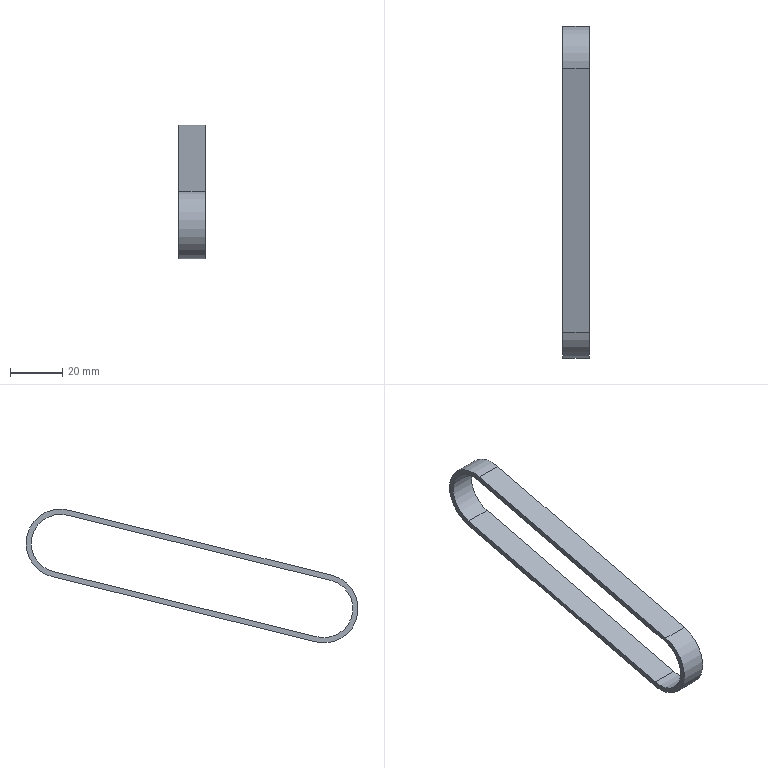Component | SolidWorks | RearConveyorLine,Width17mm-1 | 1 solid | 12 faces | box 10 x 127.47 x 51.3 mm | volume 5695 mm3 | cylinder 6 | plane 6 | commonest cylinder face diameters 22.28 x3 26.28 x3
build123d program:
from build123d import *

# Parameters (mm, degrees)
BOSS_EXTRUDE1_DEPTH = 5


with BuildPart() as part:
    # Sketch1 → Boss-Extrude1 (new, symmetric)
    with BuildSketch(Plane(origin=(0, 0, 0), x_dir=(0, 0, -1), z_dir=(1, 0, 0))):
        with BuildLine():
            Line((-52.12, 13.14), (52.12, 13.14))
            ThreePointArc((52.12, 13.14), (65.26, 0), (52.12, -13.14))
            Line((52.12, -13.14), (-52.12, -13.14))
            ThreePointArc((-52.12, -13.14), (-65.26, 0), (-52.12, 13.14))
        make_face()
        with BuildLine():
            Line((-52.12, 11.14), (52.12, 11.14))
            ThreePointArc((52.12, 11.14), (63.26, 0), (52.12, -11.14))
            Line((52.12, -11.14), (-52.12, -11.14))
            ThreePointArc((-52.12, -11.14), (-63.26, 0), (-52.12, 11.14))
        make_face(mode=Mode.SUBTRACT)
    extrude(amount=BOSS_EXTRUDE1_DEPTH, both=True)


solid = part.part

# Placed as in the assembly
solid = solid.moved(Location((-20.5, -50.596, 137.489), (103.889, 0, 180)))
STEP:
#1=COLOUR_RGB('',0.7922,0.8196,0.9333);
#2=FILL_AREA_STYLE_COLOUR('',#1);
#3=FILL_AREA_STYLE('',(#2));
#4=SURFACE_STYLE_FILL_AREA(#3);
#5=SURFACE_SIDE_STYLE('',(#4));
#6=SURFACE_STYLE_USAGE(.BOTH.,#5);
#7=PRESENTATION_STYLE_ASSIGNMENT((#6));
#8=CARTESIAN_POINT('',(-0.6102,0.1053,5.48));
#9=VERTEX_POINT('',#8);
#10=CARTESIAN_POINT('',(-0.6102,0.4258,6.011));
#11=VERTEX_POINT('',#10);
#12=CARTESIAN_POINT('',(-0.6102,-0.,5.906));
#13=DIRECTION('',(1.,0.,0.));
#14=DIRECTION('',(0.,-0.9708,-0.24));
#15=AXIS2_PLACEMENT_3D('',#12,#13,#14);
#16=CIRCLE('',#15,0.4386);
#17=EDGE_CURVE('',#9,#11,#16,.T.);
#18=ORIENTED_EDGE('',*,*,#17,.T.);
#19=CARTESIAN_POINT('',(-1.004,0.4258,6.011));
#20=VERTEX_POINT('',#19);
#21=CARTESIAN_POINT('',(-0.6102,0.4258,6.011));
#22=DIRECTION('',(-1.,0.,0.));
#23=VECTOR('',#22,39.37);
#24=LINE('',#21,#23);
#25=EDGE_CURVE('',#11,#20,#24,.T.);
#26=ORIENTED_EDGE('',*,*,#25,.T.);
#27=CARTESIAN_POINT('',(-1.004,0.1053,5.48));
#28=VERTEX_POINT('',#27);
#29=CARTESIAN_POINT('',(-1.004,-0.,5.906));
#30=DIRECTION('',(1.,0.,0.));
#31=DIRECTION('',(0.,-0.9708,-0.24));
#32=AXIS2_PLACEMENT_3D('',#29,#30,#31);
#33=CIRCLE('',#32,0.4386);
#34=EDGE_CURVE('',#28,#20,#33,.T.);
#35=ORIENTED_EDGE('',*,*,#34,.F.);
#36=CARTESIAN_POINT('',(-0.6102,0.1053,5.48));
#37=DIRECTION('',(-1.,0.,0.));
#38=VECTOR('',#37,39.37);
#39=LINE('',#36,#38);
#40=EDGE_CURVE('',#9,#28,#39,.T.);
#41=ORIENTED_EDGE('',*,*,#40,.F.);
#42=EDGE_LOOP('',(#18,#26,#35,#41));
#43=FACE_OUTER_BOUND('',#42,.T.);
#44=CARTESIAN_POINT('',(-0.6102,-0.,5.906));
#45=DIRECTION('',(-1.,0.,0.));
#46=DIRECTION('',(0.,0.9708,0.24));
#47=AXIS2_PLACEMENT_3D('',#44,#45,#46);
#48=CYLINDRICAL_SURFACE('',#47,0.4386);
#49=ADVANCED_FACE('',(#43),#48,.F.);
#50=CARTESIAN_POINT('',(-0.6102,0.5022,6.03));
#51=VERTEX_POINT('',#50);
#52=CARTESIAN_POINT('',(-0.6102,-0.1242,6.408));
#53=VERTEX_POINT('',#52);
#54=CARTESIAN_POINT('',(-0.6102,-0.,5.906));
#55=DIRECTION('',(1.,0.,0.));
#56=DIRECTION('',(0.,-0.9708,-0.24));
#57=AXIS2_PLACEMENT_3D('',#54,#55,#56);
#58=CIRCLE('',#57,0.5173);
#59=EDGE_CURVE('',#51,#53,#58,.T.);
#60=ORIENTED_EDGE('',*,*,#59,.F.);
#61=CARTESIAN_POINT('',(-1.004,0.5022,6.03));
#62=VERTEX_POINT('',#61);
#63=CARTESIAN_POINT('',(-0.6102,0.5022,6.03));
#64=DIRECTION('',(-1.,0.,0.));
#65=VECTOR('',#64,39.37);
#66=LINE('',#63,#65);
#67=EDGE_CURVE('',#51,#62,#66,.T.);
#68=ORIENTED_EDGE('',*,*,#67,.T.);
#69=CARTESIAN_POINT('',(-1.004,-0.1242,6.408));
#70=VERTEX_POINT('',#69);
#71=CARTESIAN_POINT('',(-1.004,-0.,5.906));
#72=DIRECTION('',(1.,0.,0.));
#73=DIRECTION('',(0.,-0.9708,-0.24));
#74=AXIS2_PLACEMENT_3D('',#71,#72,#73);
#75=CIRCLE('',#74,0.5173);
#76=EDGE_CURVE('',#62,#70,#75,.T.);
#77=ORIENTED_EDGE('',*,*,#76,.T.);
#78=CARTESIAN_POINT('',(-0.6102,-0.1242,6.408));
#79=DIRECTION('',(-1.,0.,0.));
#80=VECTOR('',#79,39.37);
#81=LINE('',#78,#80);
#82=EDGE_CURVE('',#53,#70,#81,.T.);
#83=ORIENTED_EDGE('',*,*,#82,.F.);
#84=EDGE_LOOP('',(#60,#68,#77,#83));
#85=FACE_OUTER_BOUND('',#84,.T.);
#86=CARTESIAN_POINT('',(-0.6102,-0.,5.906));
#87=DIRECTION('',(-1.,0.,0.));
#88=DIRECTION('',(0.,0.9708,0.24));
#89=AXIS2_PLACEMENT_3D('',#86,#87,#88);
#90=CYLINDRICAL_SURFACE('',#89,0.5173);
#91=ADVANCED_FACE('',(#85),#90,.T.);
#92=CARTESIAN_POINT('',(-0.6102,0.1242,5.403));
#93=VERTEX_POINT('',#92);
#94=CARTESIAN_POINT('',(-0.6102,-0.,5.906));
#95=DIRECTION('',(1.,0.,0.));
#96=DIRECTION('',(0.,-0.9708,-0.24));
#97=AXIS2_PLACEMENT_3D('',#94,#95,#96);
#98=CIRCLE('',#97,0.5173);
#99=EDGE_CURVE('',#93,#51,#98,.T.);
#100=ORIENTED_EDGE('',*,*,#99,.T.);
#101=ORIENTED_EDGE('',*,*,#59,.T.);
#102=CARTESIAN_POINT('',(-0.6102,-4.108,5.423));
#103=VERTEX_POINT('',#102);
#104=CARTESIAN_POINT('',(-0.6102,-0.1242,6.408));
#105=DIRECTION('',(0.,-0.9708,-0.24));
#106=VECTOR('',#105,39.37);
#107=LINE('',#104,#106);
#108=EDGE_CURVE('',#53,#103,#107,.T.);
#109=ORIENTED_EDGE('',*,*,#108,.T.);
#110=CARTESIAN_POINT('',(-0.6102,-3.86,4.418));
#111=VERTEX_POINT('',#110);
#112=CARTESIAN_POINT('',(-0.6102,-3.984,4.92));
#113=DIRECTION('',(1.,0.,0.));
#114=DIRECTION('',(0.,-0.9708,-0.24));
#115=AXIS2_PLACEMENT_3D('',#112,#113,#114);
#116=CIRCLE('',#115,0.5173);
#117=EDGE_CURVE('',#103,#111,#116,.T.);
#118=ORIENTED_EDGE('',*,*,#117,.T.);
#119=CARTESIAN_POINT('',(-0.6102,0.1242,5.403));
#120=DIRECTION('',(0.,0.9708,0.24));
#121=VECTOR('',#120,39.37);
#122=LINE('',#119,#121);
#123=EDGE_CURVE('',#111,#93,#122,.T.);
#124=ORIENTED_EDGE('',*,*,#123,.T.);
#125=EDGE_LOOP('',(#100,#101,#109,#118,#124));
#126=FACE_OUTER_BOUND('',#125,.T.);
#127=CARTESIAN_POINT('',(-0.6102,-0.1053,6.331));
#128=VERTEX_POINT('',#127);
#129=CARTESIAN_POINT('',(-0.6102,-4.089,5.346));
#130=VERTEX_POINT('',#129);
#131=CARTESIAN_POINT('',(-0.6102,-0.1053,6.331));
#132=DIRECTION('',(0.,-0.9708,-0.24));
#133=VECTOR('',#132,39.37);
#134=LINE('',#131,#133);
#135=EDGE_CURVE('',#128,#130,#134,.T.);
#136=ORIENTED_EDGE('',*,*,#135,.F.);
#137=CARTESIAN_POINT('',(-0.6102,-0.,5.906));
#138=DIRECTION('',(1.,0.,0.));
#139=DIRECTION('',(0.,-0.9708,-0.24));
#140=AXIS2_PLACEMENT_3D('',#137,#138,#139);
#141=CIRCLE('',#140,0.4386);
#142=EDGE_CURVE('',#11,#128,#141,.T.);
#143=ORIENTED_EDGE('',*,*,#142,.F.);
#144=ORIENTED_EDGE('',*,*,#17,.F.);
#145=CARTESIAN_POINT('',(-0.6102,-3.879,4.495));
#146=VERTEX_POINT('',#145);
#147=CARTESIAN_POINT('',(-0.6102,0.1053,5.48));
#148=DIRECTION('',(0.,0.9708,0.24));
#149=VECTOR('',#148,39.37);
#150=LINE('',#147,#149);
#151=EDGE_CURVE('',#146,#9,#150,.T.);
#152=ORIENTED_EDGE('',*,*,#151,.F.);
#153=CARTESIAN_POINT('',(-0.6102,-3.984,4.92));
#154=DIRECTION('',(1.,0.,0.));
#155=DIRECTION('',(0.,-0.9708,-0.24));
#156=AXIS2_PLACEMENT_3D('',#153,#154,#155);
#157=CIRCLE('',#156,0.4386);
#158=EDGE_CURVE('',#130,#146,#157,.T.);
#159=ORIENTED_EDGE('',*,*,#158,.F.);
#160=EDGE_LOOP('',(#136,#143,#144,#152,#159));
#161=FACE_BOUND('',#160,.T.);
#162=CARTESIAN_POINT('',(-0.6102,-0.,5.906));
#163=DIRECTION('',(1.,0.,0.));
#164=DIRECTION('',(0.,-0.9708,-0.24));
#165=AXIS2_PLACEMENT_3D('',#162,#163,#164);
#166=PLANE('',#165);
#167=ADVANCED_FACE('',(#126,#161),#166,.T.);
#168=CARTESIAN_POINT('',(-1.004,0.1242,5.403));
#169=VERTEX_POINT('',#168);
#170=CARTESIAN_POINT('',(-1.004,-0.,5.906));
#171=DIRECTION('',(1.,0.,0.));
#172=DIRECTION('',(0.,-0.9708,-0.24));
#173=AXIS2_PLACEMENT_3D('',#170,#171,#172);
#174=CIRCLE('',#173,0.5173);
#175=EDGE_CURVE('',#169,#62,#174,.T.);
#176=ORIENTED_EDGE('',*,*,#175,.F.);
#177=CARTESIAN_POINT('',(-1.004,-3.86,4.418));
#178=VERTEX_POINT('',#177);
#179=CARTESIAN_POINT('',(-1.004,0.1242,5.403));
#180=DIRECTION('',(0.,0.9708,0.24));
#181=VECTOR('',#180,39.37);
#182=LINE('',#179,#181);
#183=EDGE_CURVE('',#178,#169,#182,.T.);
#184=ORIENTED_EDGE('',*,*,#183,.F.);
#185=CARTESIAN_POINT('',(-1.004,-4.108,5.423));
#186=VERTEX_POINT('',#185);
#187=CARTESIAN_POINT('',(-1.004,-3.984,4.92));
#188=DIRECTION('',(1.,0.,0.));
#189=DIRECTION('',(0.,-0.9708,-0.24));
#190=AXIS2_PLACEMENT_3D('',#187,#188,#189);
#191=CIRCLE('',#190,0.5173);
#192=EDGE_CURVE('',#186,#178,#191,.T.);
#193=ORIENTED_EDGE('',*,*,#192,.F.);
#194=CARTESIAN_POINT('',(-1.004,-0.1242,6.408));
#195=DIRECTION('',(0.,-0.9708,-0.24));
#196=VECTOR('',#195,39.37);
#197=LINE('',#194,#196);
#198=EDGE_CURVE('',#70,#186,#197,.T.);
#199=ORIENTED_EDGE('',*,*,#198,.F.);
#200=ORIENTED_EDGE('',*,*,#76,.F.);
#201=EDGE_LOOP('',(#176,#184,#193,#199,#200));
#202=FACE_OUTER_BOUND('',#201,.T.);
#203=ORIENTED_EDGE('',*,*,#34,.T.);
#204=CARTESIAN_POINT('',(-1.004,-0.1053,6.331));
#205=VERTEX_POINT('',#204);
#206=CARTESIAN_POINT('',(-1.004,-0.,5.906));
#207=DIRECTION('',(1.,0.,0.));
#208=DIRECTION('',(0.,-0.9708,-0.24));
#209=AXIS2_PLACEMENT_3D('',#206,#207,#208);
#210=CIRCLE('',#209,0.4386);
#211=EDGE_CURVE('',#20,#205,#210,.T.);
#212=ORIENTED_EDGE('',*,*,#211,.T.);
#213=CARTESIAN_POINT('',(-1.004,-4.089,5.346));
#214=VERTEX_POINT('',#213);
#215=CARTESIAN_POINT('',(-1.004,-0.1053,6.331));
#216=DIRECTION('',(0.,-0.9708,-0.24));
#217=VECTOR('',#216,39.37);
#218=LINE('',#215,#217);
#219=EDGE_CURVE('',#205,#214,#218,.T.);
#220=ORIENTED_EDGE('',*,*,#219,.T.);
#221=CARTESIAN_POINT('',(-1.004,-3.879,4.495));
#222=VERTEX_POINT('',#221);
#223=CARTESIAN_POINT('',(-1.004,-3.984,4.92));
#224=DIRECTION('',(1.,0.,0.));
#225=DIRECTION('',(0.,-0.9708,-0.24));
#226=AXIS2_PLACEMENT_3D('',#223,#224,#225);
#227=CIRCLE('',#226,0.4386);
#228=EDGE_CURVE('',#214,#222,#227,.T.);
#229=ORIENTED_EDGE('',*,*,#228,.T.);
#230=CARTESIAN_POINT('',(-1.004,0.1053,5.48));
#231=DIRECTION('',(0.,0.9708,0.24));
#232=VECTOR('',#231,39.37);
#233=LINE('',#230,#232);
#234=EDGE_CURVE('',#222,#28,#233,.T.);
#235=ORIENTED_EDGE('',*,*,#234,.T.);
#236=EDGE_LOOP('',(#203,#212,#220,#229,#235));
#237=FACE_BOUND('',#236,.T.);
#238=CARTESIAN_POINT('',(-1.004,-0.,5.906));
#239=DIRECTION('',(1.,0.,0.));
#240=DIRECTION('',(0.,-0.9708,-0.24));
#241=AXIS2_PLACEMENT_3D('',#238,#239,#240);
#242=PLANE('',#241);
#243=ADVANCED_FACE('',(#202,#237),#242,.F.);
#244=ORIENTED_EDGE('',*,*,#67,.F.);
#245=ORIENTED_EDGE('',*,*,#99,.F.);
#246=CARTESIAN_POINT('',(-0.6102,0.1242,5.403));
#247=DIRECTION('',(-1.,0.,0.));
#248=VECTOR('',#247,39.37);
#249=LINE('',#246,#248);
#250=EDGE_CURVE('',#93,#169,#249,.T.);
#251=ORIENTED_EDGE('',*,*,#250,.T.);
#252=ORIENTED_EDGE('',*,*,#175,.T.);
#253=EDGE_LOOP('',(#244,#245,#251,#252));
#254=FACE_OUTER_BOUND('',#253,.T.);
#255=CARTESIAN_POINT('',(-0.6102,-0.,5.906));
#256=DIRECTION('',(-1.,0.,0.));
#257=DIRECTION('',(0.,0.9708,0.24));
#258=AXIS2_PLACEMENT_3D('',#255,#256,#257);
#259=CYLINDRICAL_SURFACE('',#258,0.5173);
#260=ADVANCED_FACE('',(#254),#259,.T.);
#261=ORIENTED_EDGE('',*,*,#198,.T.);
#262=CARTESIAN_POINT('',(-0.6102,-4.108,5.423));
#263=DIRECTION('',(-1.,0.,0.));
#264=VECTOR('',#263,39.37);
#265=LINE('',#262,#264);
#266=EDGE_CURVE('',#103,#186,#265,.T.);
#267=ORIENTED_EDGE('',*,*,#266,.F.);
#268=ORIENTED_EDGE('',*,*,#108,.F.);
#269=ORIENTED_EDGE('',*,*,#82,.T.);
#270=EDGE_LOOP('',(#261,#267,#268,#269));
#271=FACE_OUTER_BOUND('',#270,.T.);
#272=CARTESIAN_POINT('',(-0.6102,-0.1242,6.408));
#273=DIRECTION('',(0.,0.24,-0.9708));
#274=DIRECTION('',(0.,0.9708,0.24));
#275=AXIS2_PLACEMENT_3D('',#272,#273,#274);
#276=PLANE('',#275);
#277=ADVANCED_FACE('',(#271),#276,.F.);
#278=ORIENTED_EDGE('',*,*,#192,.T.);
#279=CARTESIAN_POINT('',(-0.6102,-3.86,4.418));
#280=DIRECTION('',(-1.,0.,0.));
#281=VECTOR('',#280,39.37);
#282=LINE('',#279,#281);
#283=EDGE_CURVE('',#111,#178,#282,.T.);
#284=ORIENTED_EDGE('',*,*,#283,.F.);
#285=ORIENTED_EDGE('',*,*,#117,.F.);
#286=ORIENTED_EDGE('',*,*,#266,.T.);
#287=EDGE_LOOP('',(#278,#284,#285,#286));
#288=FACE_OUTER_BOUND('',#287,.T.);
#289=CARTESIAN_POINT('',(-0.6102,-3.984,4.92));
#290=DIRECTION('',(-1.,0.,0.));
#291=DIRECTION('',(0.,0.9708,0.24));
#292=AXIS2_PLACEMENT_3D('',#289,#290,#291);
#293=CYLINDRICAL_SURFACE('',#292,0.5173);
#294=ADVANCED_FACE('',(#288),#293,.T.);
#295=ORIENTED_EDGE('',*,*,#183,.T.);
#296=ORIENTED_EDGE('',*,*,#250,.F.);
#297=ORIENTED_EDGE('',*,*,#123,.F.);
#298=ORIENTED_EDGE('',*,*,#283,.T.);
#299=EDGE_LOOP('',(#295,#296,#297,#298));
#300=FACE_OUTER_BOUND('',#299,.T.);
#301=CARTESIAN_POINT('',(-0.6102,0.1242,5.403));
#302=DIRECTION('',(0.,-0.24,0.9708));
#303=DIRECTION('',(0.,-0.9708,-0.24));
#304=AXIS2_PLACEMENT_3D('',#301,#302,#303);
#305=PLANE('',#304);
#306=ADVANCED_FACE('',(#300),#305,.F.);
#307=ORIENTED_EDGE('',*,*,#25,.F.);
#308=ORIENTED_EDGE('',*,*,#142,.T.);
#309=CARTESIAN_POINT('',(-0.6102,-0.1053,6.331));
#310=DIRECTION('',(-1.,0.,0.));
#311=VECTOR('',#310,39.37);
#312=LINE('',#309,#311);
#313=EDGE_CURVE('',#128,#205,#312,.T.);
#314=ORIENTED_EDGE('',*,*,#313,.T.);
#315=ORIENTED_EDGE('',*,*,#211,.F.);
#316=EDGE_LOOP('',(#307,#308,#314,#315));
#317=FACE_OUTER_BOUND('',#316,.T.);
#318=CARTESIAN_POINT('',(-0.6102,-0.,5.906));
#319=DIRECTION('',(-1.,0.,0.));
#320=DIRECTION('',(0.,0.9708,0.24));
#321=AXIS2_PLACEMENT_3D('',#318,#319,#320);
#322=CYLINDRICAL_SURFACE('',#321,0.4386);
#323=ADVANCED_FACE('',(#317),#322,.F.);
#324=ORIENTED_EDGE('',*,*,#219,.F.);
#325=ORIENTED_EDGE('',*,*,#313,.F.);
#326=ORIENTED_EDGE('',*,*,#135,.T.);
#327=CARTESIAN_POINT('',(-0.6102,-4.089,5.346));
#328=DIRECTION('',(-1.,0.,0.));
#329=VECTOR('',#328,39.37);
#330=LINE('',#327,#329);
#331=EDGE_CURVE('',#130,#214,#330,.T.);
#332=ORIENTED_EDGE('',*,*,#331,.T.);
#333=EDGE_LOOP('',(#324,#325,#326,#332));
#334=FACE_OUTER_BOUND('',#333,.T.);
#335=CARTESIAN_POINT('',(-0.6102,-0.1053,6.331));
#336=DIRECTION('',(0.,0.24,-0.9708));
#337=DIRECTION('',(0.,0.9708,0.24));
#338=AXIS2_PLACEMENT_3D('',#335,#336,#337);
#339=PLANE('',#338);
#340=ADVANCED_FACE('',(#334),#339,.T.);
#341=ORIENTED_EDGE('',*,*,#228,.F.);
#342=ORIENTED_EDGE('',*,*,#331,.F.);
#343=ORIENTED_EDGE('',*,*,#158,.T.);
#344=CARTESIAN_POINT('',(-0.6102,-3.879,4.495));
#345=DIRECTION('',(-1.,0.,0.));
#346=VECTOR('',#345,39.37);
#347=LINE('',#344,#346);
#348=EDGE_CURVE('',#146,#222,#347,.T.);
#349=ORIENTED_EDGE('',*,*,#348,.T.);
#350=EDGE_LOOP('',(#341,#342,#343,#349));
#351=FACE_OUTER_BOUND('',#350,.T.);
#352=CARTESIAN_POINT('',(-0.6102,-3.984,4.92));
#353=DIRECTION('',(-1.,0.,0.));
#354=DIRECTION('',(0.,0.9708,0.24));
#355=AXIS2_PLACEMENT_3D('',#352,#353,#354);
#356=CYLINDRICAL_SURFACE('',#355,0.4386);
#357=ADVANCED_FACE('',(#351),#356,.F.);
#358=ORIENTED_EDGE('',*,*,#234,.F.);
#359=ORIENTED_EDGE('',*,*,#348,.F.);
#360=ORIENTED_EDGE('',*,*,#151,.T.);
#361=ORIENTED_EDGE('',*,*,#40,.T.);
#362=EDGE_LOOP('',(#358,#359,#360,#361));
#363=FACE_OUTER_BOUND('',#362,.T.);
#364=CARTESIAN_POINT('',(-0.6102,0.1053,5.48));
#365=DIRECTION('',(0.,-0.24,0.9708));
#366=DIRECTION('',(0.,-0.9708,-0.24));
#367=AXIS2_PLACEMENT_3D('',#364,#365,#366);
#368=PLANE('',#367);
#369=ADVANCED_FACE('',(#363),#368,.T.);
#370=CLOSED_SHELL('',(#49,#91,#167,#243,#260,#277,#294,#306,#323,#340,#357,#369));
#371=MANIFOLD_SOLID_BREP('',#370);
#372=STYLED_ITEM('',(#7),#371);
#373=PRESENTATION_LAYER_ASSIGNMENT('','',(#372));
#374=(LENGTH_UNIT()NAMED_UNIT(*)SI_UNIT($,.METRE.));
#375=LENGTH_MEASURE_WITH_UNIT(LENGTH_MEASURE(0.0254),#374);
#376=DIMENSIONAL_EXPONENTS(1.,0.,0.,0.,0.,0.,0.);
#377=(CONVERSION_BASED_UNIT('',#375)LENGTH_UNIT()NAMED_UNIT(#376));
#378=UNCERTAINTY_MEASURE_WITH_UNIT(LENGTH_MEASURE(0.00001),#377,'','');
#379=(NAMED_UNIT(*)PLANE_ANGLE_UNIT()SI_UNIT($,.RADIAN.));
#380=(NAMED_UNIT(*)SI_UNIT($,.STERADIAN.)SOLID_ANGLE_UNIT());
#381=(GEOMETRIC_REPRESENTATION_CONTEXT(3)GLOBAL_UNCERTAINTY_ASSIGNED_CONTEXT((#378))GLOBAL_UNIT_ASSIGNED_CONTEXT((#377,#379,#380))REPRESENTATION_CONTEXT('',''));
#382=MECHANICAL_DESIGN_GEOMETRIC_PRESENTATION_REPRESENTATION('',(#372),#381);
#383=CARTESIAN_POINT('',(0.,0.,0.));
#384=DIRECTION('',(0.,0.,1.));
#385=DIRECTION('',(1.,0.,0.));
#386=AXIS2_PLACEMENT_3D('',#383,#384,#385);
#387=(LENGTH_UNIT()NAMED_UNIT(*)SI_UNIT($,.METRE.));
#388=LENGTH_MEASURE_WITH_UNIT(LENGTH_MEASURE(0.0254),#387);
#389=DIMENSIONAL_EXPONENTS(1.,0.,0.,0.,0.,0.,0.);
#390=(CONVERSION_BASED_UNIT('',#388)LENGTH_UNIT()NAMED_UNIT(#389));
#391=UNCERTAINTY_MEASURE_WITH_UNIT(LENGTH_MEASURE(0.00001),#390,'','');
#392=(NAMED_UNIT(*)PLANE_ANGLE_UNIT()SI_UNIT($,.RADIAN.));
#393=(NAMED_UNIT(*)SI_UNIT($,.STERADIAN.)SOLID_ANGLE_UNIT());
#394=(GEOMETRIC_REPRESENTATION_CONTEXT(3)GLOBAL_UNCERTAINTY_ASSIGNED_CONTEXT((#391))GLOBAL_UNIT_ASSIGNED_CONTEXT((#390,#392,#393))REPRESENTATION_CONTEXT('',''));
#395=ADVANCED_BREP_SHAPE_REPRESENTATION('',(#371,#386),#394);